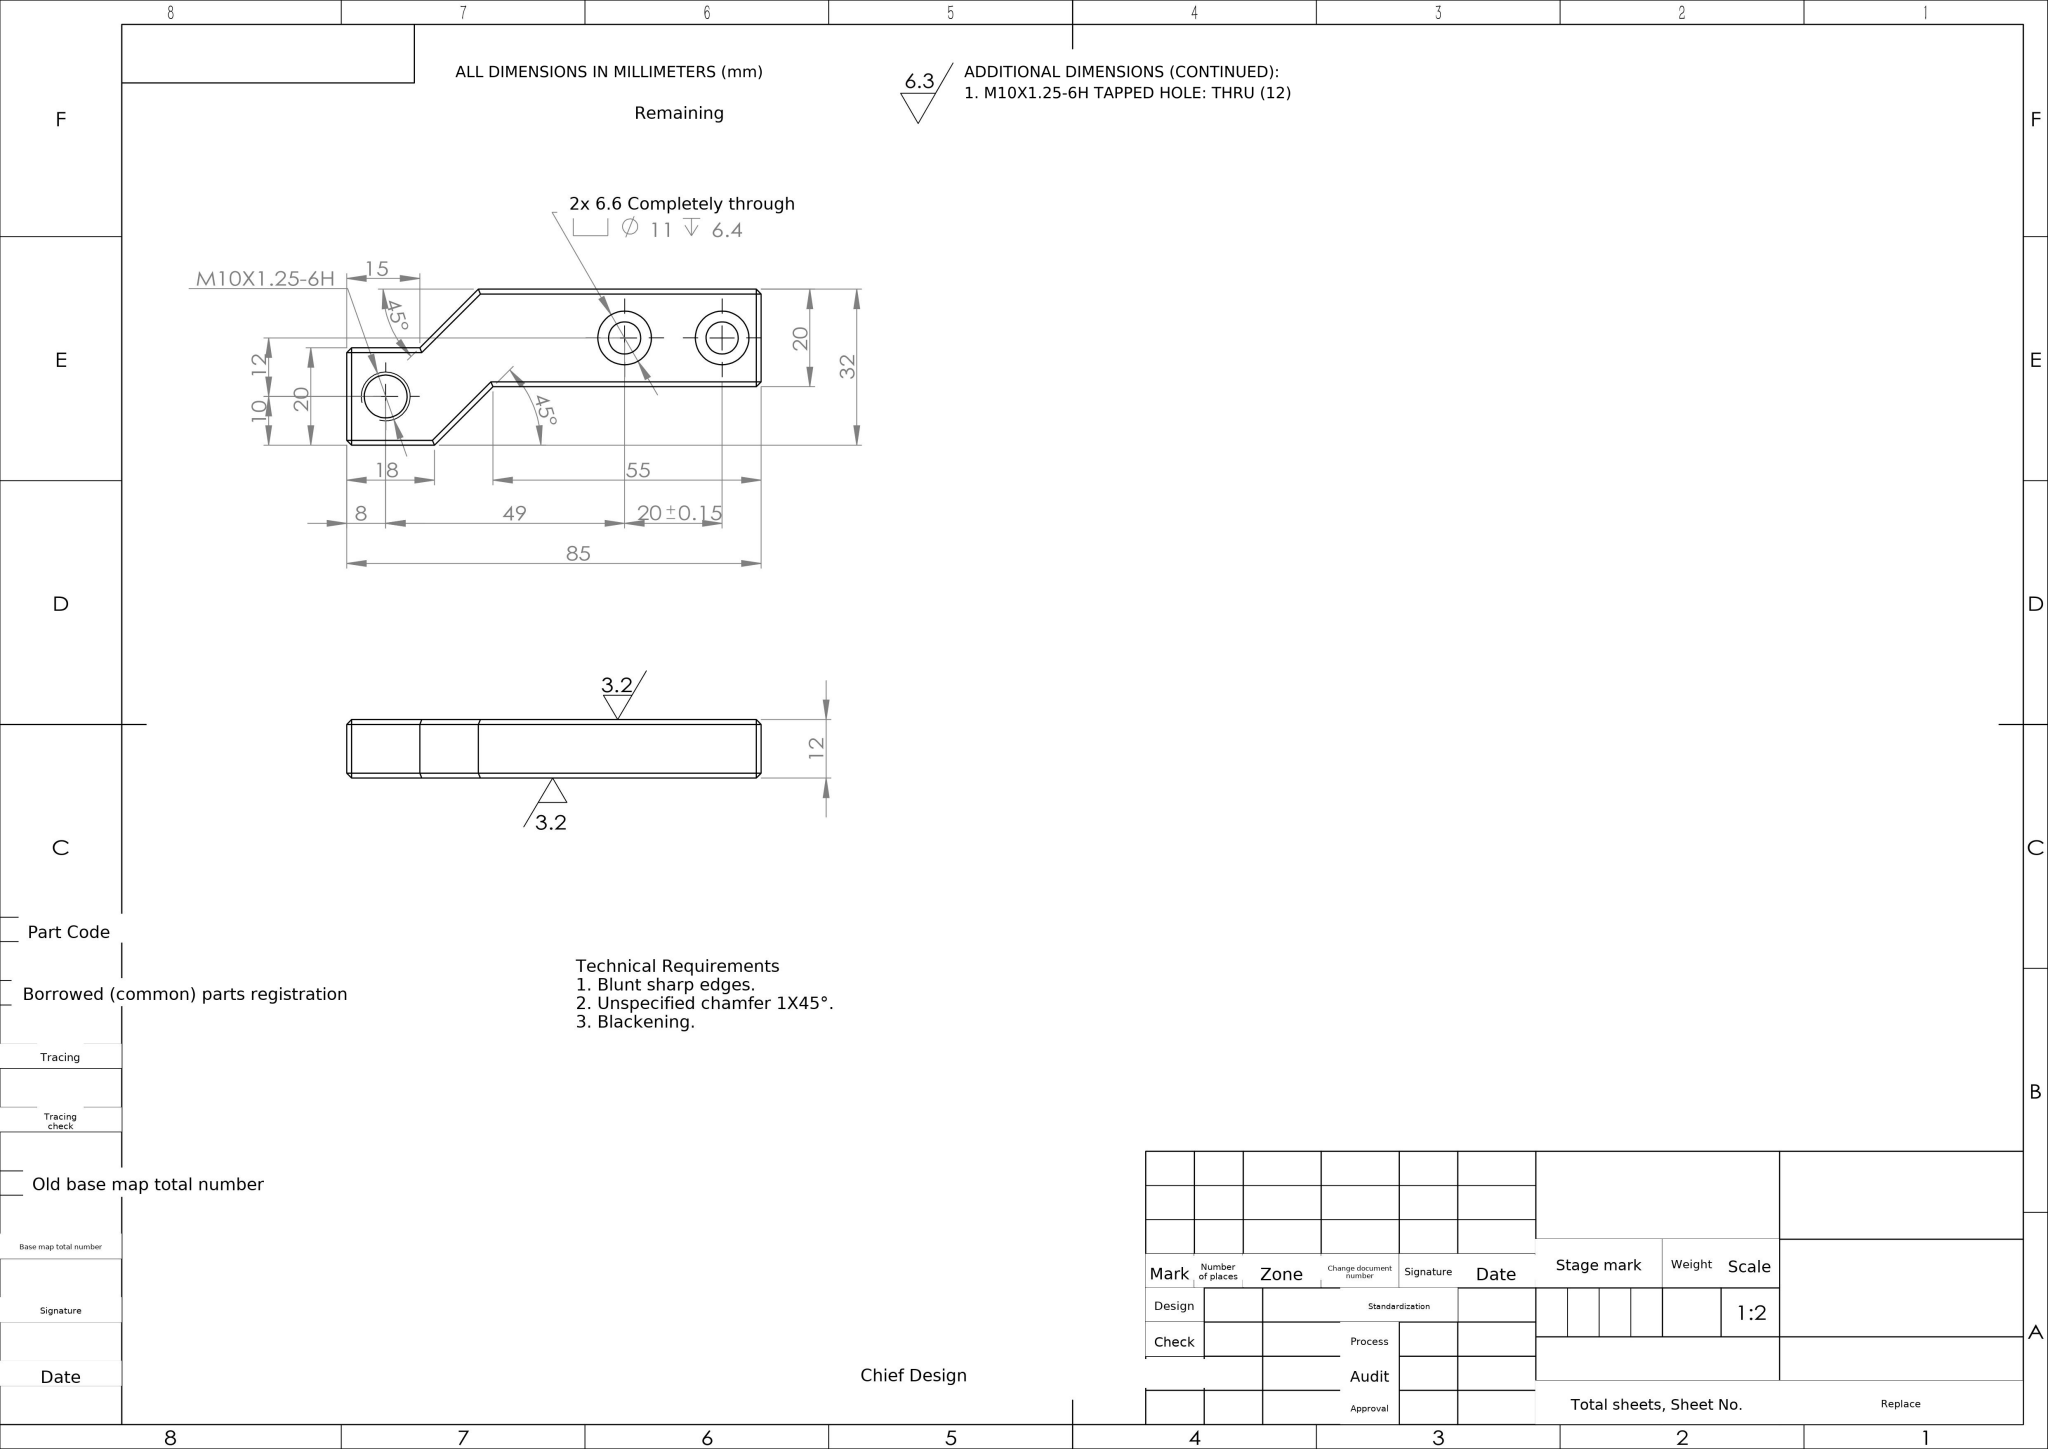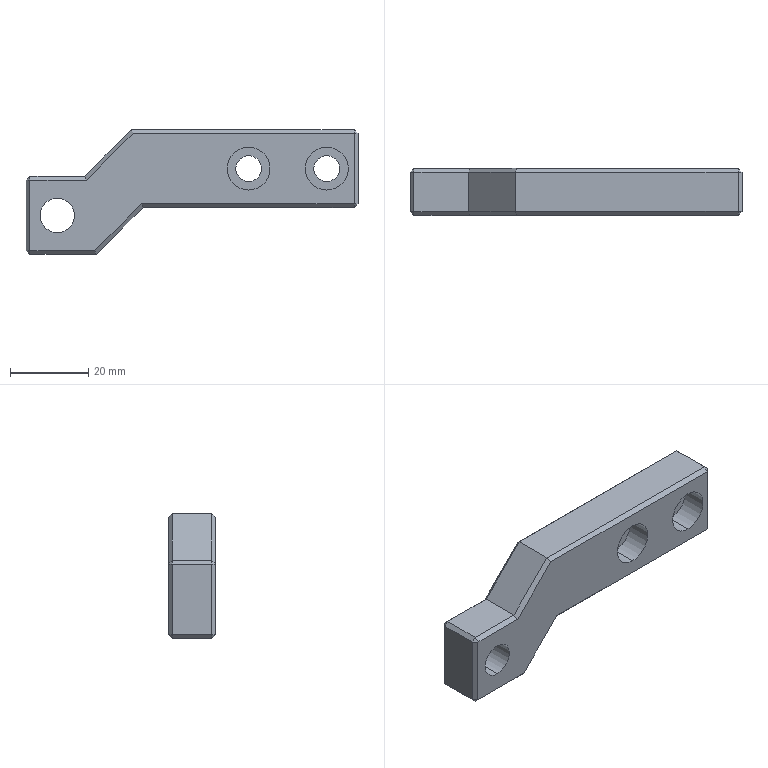Part | NX | mm | 1 solid | 50 faces | box 85 x 12 x 32 mm | volume 18264 mm3 | plane 40 | cylinder 10 | commonest cylinder face diameters 11 x4 6.6 x4 8.8 x2